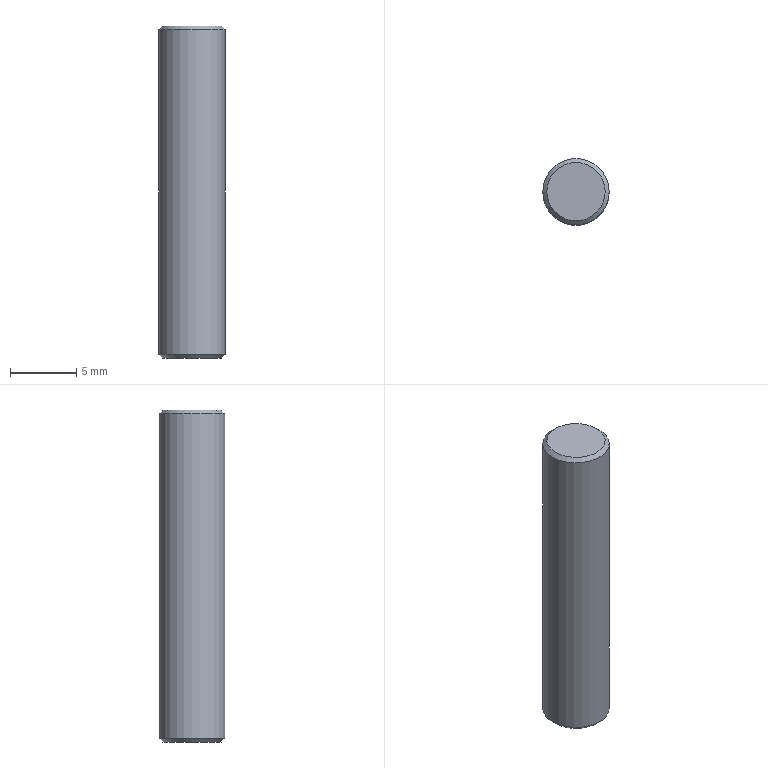Component | NX | DOWEL_PIN | 1 solid | 5 faces | box 5 x 5 x 25 mm | volume 490 mm3 | plane 2 | cone 2 | cylinder 1 | commonest cylinder face diameters 5 x1
STEP:
#1=CARTESIAN_POINT('',(0.,0.,0.));
#2=DIRECTION('',(0.,0.,1.));
#3=DIRECTION('',(1.,0.,0.));
#4=AXIS2_PLACEMENT_3D('',#1,#2,#3);
#5=CARTESIAN_POINT('',(96.2,25.,-225.));
#6=VERTEX_POINT('',#5);
#7=CARTESIAN_POINT('',(94.,25.,-225.));
#8=DIRECTION('',(0.,0.,1.));
#9=DIRECTION('',(1.,0.,0.));
#10=AXIS2_PLACEMENT_3D('',#7,#8,#9);
#11=CIRCLE('',#10,2.2);
#12=CARTESIAN_POINT('',(94.,25.,-225.));
#13=DIRECTION('',(0.,0.,1.));
#14=DIRECTION('',(1.,0.,0.));
#15=AXIS2_PLACEMENT_3D('',#12,#13,#14);
#16=PLANE('',#15);
#17=CARTESIAN_POINT('',(0.,0.));
#18=DIRECTION('',(1.,0.));
#19=AXIS2_PLACEMENT_2D('',#17,#18);
#20=CIRCLE('',#19,2.2);
#21=(GEOMETRIC_REPRESENTATION_CONTEXT(2)PARAMETRIC_REPRESENTATION_CONTEXT()REPRESENTATION_CONTEXT('',''));
#22=DEFINITIONAL_REPRESENTATION('',(#20),#21);
#23=PCURVE('',#16,#22);
#24=CARTESIAN_POINT('',(94.,25.,-225.3));
#25=DIRECTION('',(0.,0.,-1.));
#26=DIRECTION('',(-1.,0.,0.));
#27=AXIS2_PLACEMENT_3D('',#24,#25,#26);
#28=CONICAL_SURFACE('',#27,2.5,0.7854);
#29=CARTESIAN_POINT('',(9.425,-0.3));
#30=DIRECTION('',(-1.,0.));
#31=VECTOR('',#30,1.);
#32=LINE('',#29,#31);
#33=(GEOMETRIC_REPRESENTATION_CONTEXT(2)PARAMETRIC_REPRESENTATION_CONTEXT()REPRESENTATION_CONTEXT('',''));
#34=DEFINITIONAL_REPRESENTATION('',(#32),#33);
#35=PCURVE('',#28,#34);
#36=SURFACE_CURVE('',#11,(#23,#35),.PCURVE_S1.);
#37=EDGE_CURVE('',#6,#6,#36,.T.);
#38=ORIENTED_EDGE('',*,*,#37,.T.);
#39=EDGE_LOOP('',(#38));
#40=FACE_BOUND('',#39,.T.);
#41=ADVANCED_FACE('',(#40),#16,.T.);
#42=CARTESIAN_POINT('',(91.8,25.,-250.));
#43=VERTEX_POINT('',#42);
#44=CARTESIAN_POINT('',(94.,25.,-250.));
#45=DIRECTION('',(0.,0.,-1.));
#46=DIRECTION('',(-1.,0.,0.));
#47=AXIS2_PLACEMENT_3D('',#44,#45,#46);
#48=CIRCLE('',#47,2.2);
#49=CARTESIAN_POINT('',(94.,25.,-250.));
#50=DIRECTION('',(0.,0.,-1.));
#51=DIRECTION('',(-1.,0.,0.));
#52=AXIS2_PLACEMENT_3D('',#49,#50,#51);
#53=PLANE('',#52);
#54=CARTESIAN_POINT('',(0.,0.));
#55=DIRECTION('',(1.,0.));
#56=AXIS2_PLACEMENT_2D('',#54,#55);
#57=CIRCLE('',#56,2.2);
#58=(GEOMETRIC_REPRESENTATION_CONTEXT(2)PARAMETRIC_REPRESENTATION_CONTEXT()REPRESENTATION_CONTEXT('',''));
#59=DEFINITIONAL_REPRESENTATION('',(#57),#58);
#60=PCURVE('',#53,#59);
#61=CARTESIAN_POINT('',(94.,25.,-249.7));
#62=DIRECTION('',(0.,0.,1.));
#63=DIRECTION('',(1.,0.,0.));
#64=AXIS2_PLACEMENT_3D('',#61,#62,#63);
#65=CONICAL_SURFACE('',#64,2.5,0.7854);
#66=CARTESIAN_POINT('',(9.425,-0.3));
#67=DIRECTION('',(-1.,0.));
#68=VECTOR('',#67,1.);
#69=LINE('',#66,#68);
#70=(GEOMETRIC_REPRESENTATION_CONTEXT(2)PARAMETRIC_REPRESENTATION_CONTEXT()REPRESENTATION_CONTEXT('',''));
#71=DEFINITIONAL_REPRESENTATION('',(#69),#70);
#72=PCURVE('',#65,#71);
#73=SURFACE_CURVE('',#48,(#60,#72),.PCURVE_S1.);
#74=EDGE_CURVE('',#43,#43,#73,.T.);
#75=ORIENTED_EDGE('',*,*,#74,.T.);
#76=EDGE_LOOP('',(#75));
#77=FACE_BOUND('',#76,.T.);
#78=ADVANCED_FACE('',(#77),#53,.T.);
#79=CARTESIAN_POINT('',(91.5,25.,-249.7));
#80=VERTEX_POINT('',#79);
#81=CARTESIAN_POINT('',(96.5,25.,-249.7));
#82=VERTEX_POINT('',#81);
#83=CARTESIAN_POINT('',(94.,25.,-249.7));
#84=DIRECTION('',(0.,0.,1.));
#85=DIRECTION('',(-1.,0.,0.));
#86=AXIS2_PLACEMENT_3D('',#83,#84,#85);
#87=CIRCLE('',#86,2.5);
#88=CARTESIAN_POINT('',(94.,25.,-250.));
#89=DIRECTION('',(0.,0.,1.));
#90=DIRECTION('',(1.,0.,0.));
#91=AXIS2_PLACEMENT_3D('',#88,#89,#90);
#92=CYLINDRICAL_SURFACE('',#91,2.5);
#93=CARTESIAN_POINT('',(3.142,0.3));
#94=DIRECTION('',(1.,0.));
#95=VECTOR('',#94,1.);
#96=LINE('',#93,#95);
#97=(GEOMETRIC_REPRESENTATION_CONTEXT(2)PARAMETRIC_REPRESENTATION_CONTEXT()REPRESENTATION_CONTEXT('',''));
#98=DEFINITIONAL_REPRESENTATION('',(#96),#97);
#99=PCURVE('',#92,#98);
#100=CARTESIAN_POINT('',(3.142,0.));
#101=DIRECTION('',(1.,0.));
#102=VECTOR('',#101,1.);
#103=LINE('',#100,#102);
#104=(GEOMETRIC_REPRESENTATION_CONTEXT(2)PARAMETRIC_REPRESENTATION_CONTEXT()REPRESENTATION_CONTEXT('',''));
#105=DEFINITIONAL_REPRESENTATION('',(#103),#104);
#106=PCURVE('',#65,#105);
#107=SURFACE_CURVE('',#87,(#99,#106),.PCURVE_S1.);
#108=EDGE_CURVE('',#80,#82,#107,.T.);
#109=ORIENTED_EDGE('',*,*,#108,.T.);
#110=CARTESIAN_POINT('',(96.5,25.,-225.3));
#111=VERTEX_POINT('',#110);
#112=CARTESIAN_POINT('',(96.5,25.,-249.7));
#113=CARTESIAN_POINT('',(96.5,25.,-225.3));
#114=B_SPLINE_CURVE_WITH_KNOTS('',1,(#112,#113),.UNSPECIFIED.,.F.,.F.,(2,2),(0.3,24.7),.PIECEWISE_BEZIER_KNOTS.);
#115=CARTESIAN_POINT('',(6.283,0.));
#116=DIRECTION('',(0.,1.));
#117=VECTOR('',#116,1.);
#118=LINE('',#115,#117);
#119=(GEOMETRIC_REPRESENTATION_CONTEXT(2)PARAMETRIC_REPRESENTATION_CONTEXT()REPRESENTATION_CONTEXT('',''));
#120=DEFINITIONAL_REPRESENTATION('',(#118),#119);
#121=PCURVE('',#92,#120);
#122=CARTESIAN_POINT('',(0.,0.));
#123=DIRECTION('',(0.,1.));
#124=VECTOR('',#123,1.);
#125=LINE('',#122,#124);
#126=(GEOMETRIC_REPRESENTATION_CONTEXT(2)PARAMETRIC_REPRESENTATION_CONTEXT()REPRESENTATION_CONTEXT('',''));
#127=DEFINITIONAL_REPRESENTATION('',(#125),#126);
#128=PCURVE('',#92,#127);
#129=SEAM_CURVE('',#114,(#121,#128),.PCURVE_S1.);
#130=EDGE_CURVE('',#82,#111,#129,.T.);
#131=ORIENTED_EDGE('',*,*,#130,.T.);
#132=CARTESIAN_POINT('',(94.,25.,-225.3));
#133=DIRECTION('',(0.,0.,-1.));
#134=DIRECTION('',(1.,0.,0.));
#135=AXIS2_PLACEMENT_3D('',#132,#133,#134);
#136=CIRCLE('',#135,2.5);
#137=CARTESIAN_POINT('',(6.283,24.7));
#138=DIRECTION('',(-1.,0.));
#139=VECTOR('',#138,1.);
#140=LINE('',#137,#139);
#141=(GEOMETRIC_REPRESENTATION_CONTEXT(2)PARAMETRIC_REPRESENTATION_CONTEXT()REPRESENTATION_CONTEXT('',''));
#142=DEFINITIONAL_REPRESENTATION('',(#140),#141);
#143=PCURVE('',#92,#142);
#144=CARTESIAN_POINT('',(3.142,0.));
#145=DIRECTION('',(1.,0.));
#146=VECTOR('',#145,1.);
#147=LINE('',#144,#146);
#148=(GEOMETRIC_REPRESENTATION_CONTEXT(2)PARAMETRIC_REPRESENTATION_CONTEXT()REPRESENTATION_CONTEXT('',''));
#149=DEFINITIONAL_REPRESENTATION('',(#147),#148);
#150=PCURVE('',#28,#149);
#151=SURFACE_CURVE('',#136,(#143,#150),.PCURVE_S1.);
#152=EDGE_CURVE('',#111,#111,#151,.T.);
#153=ORIENTED_EDGE('',*,*,#152,.T.);
#154=ORIENTED_EDGE('',*,*,#130,.F.);
#155=CARTESIAN_POINT('',(94.,25.,-249.7));
#156=DIRECTION('',(0.,0.,1.));
#157=DIRECTION('',(-1.,0.,0.));
#158=AXIS2_PLACEMENT_3D('',#155,#156,#157);
#159=CIRCLE('',#158,2.5);
#160=CARTESIAN_POINT('',(-3.142,0.3));
#161=DIRECTION('',(1.,0.));
#162=VECTOR('',#161,1.);
#163=LINE('',#160,#162);
#164=(GEOMETRIC_REPRESENTATION_CONTEXT(2)PARAMETRIC_REPRESENTATION_CONTEXT()REPRESENTATION_CONTEXT('',''));
#165=DEFINITIONAL_REPRESENTATION('',(#163),#164);
#166=PCURVE('',#92,#165);
#167=CARTESIAN_POINT('',(3.142,0.));
#168=DIRECTION('',(1.,0.));
#169=VECTOR('',#168,1.);
#170=LINE('',#167,#169);
#171=(GEOMETRIC_REPRESENTATION_CONTEXT(2)PARAMETRIC_REPRESENTATION_CONTEXT()REPRESENTATION_CONTEXT('',''));
#172=DEFINITIONAL_REPRESENTATION('',(#170),#171);
#173=PCURVE('',#65,#172);
#174=SURFACE_CURVE('',#159,(#166,#173),.PCURVE_S1.);
#175=EDGE_CURVE('',#82,#80,#174,.T.);
#176=ORIENTED_EDGE('',*,*,#175,.T.);
#177=EDGE_LOOP('',(#109,#131,#153,#154,#176));
#178=FACE_BOUND('',#177,.T.);
#179=ADVANCED_FACE('',(#178),#92,.T.);
#180=ORIENTED_EDGE('',*,*,#74,.F.);
#181=CARTESIAN_POINT('',(91.8,25.,-250.));
#182=CARTESIAN_POINT('',(91.5,25.,-249.7));
#183=B_SPLINE_CURVE_WITH_KNOTS('',1,(#181,#182),.UNSPECIFIED.,.F.,.F.,(2,2),(-0.4243,0.),.PIECEWISE_BEZIER_KNOTS.);
#184=CARTESIAN_POINT('',(9.425,0.));
#185=DIRECTION('',(0.,1.));
#186=VECTOR('',#185,1.);
#187=LINE('',#184,#186);
#188=(GEOMETRIC_REPRESENTATION_CONTEXT(2)PARAMETRIC_REPRESENTATION_CONTEXT()REPRESENTATION_CONTEXT('',''));
#189=DEFINITIONAL_REPRESENTATION('',(#187),#188);
#190=PCURVE('',#65,#189);
#191=CARTESIAN_POINT('',(3.142,0.));
#192=DIRECTION('',(0.,1.));
#193=VECTOR('',#192,1.);
#194=LINE('',#191,#193);
#195=(GEOMETRIC_REPRESENTATION_CONTEXT(2)PARAMETRIC_REPRESENTATION_CONTEXT()REPRESENTATION_CONTEXT('',''));
#196=DEFINITIONAL_REPRESENTATION('',(#194),#195);
#197=PCURVE('',#65,#196);
#198=SEAM_CURVE('',#183,(#190,#197),.PCURVE_S1.);
#199=EDGE_CURVE('',#43,#80,#198,.T.);
#200=ORIENTED_EDGE('',*,*,#199,.T.);
#201=ORIENTED_EDGE('',*,*,#175,.F.);
#202=ORIENTED_EDGE('',*,*,#108,.F.);
#203=ORIENTED_EDGE('',*,*,#199,.F.);
#204=EDGE_LOOP('',(#180,#200,#201,#202,#203));
#205=FACE_BOUND('',#204,.T.);
#206=ADVANCED_FACE('',(#205),#65,.T.);
#207=ORIENTED_EDGE('',*,*,#37,.F.);
#208=CARTESIAN_POINT('',(96.2,25.,-225.));
#209=CARTESIAN_POINT('',(96.5,25.,-225.3));
#210=B_SPLINE_CURVE_WITH_KNOTS('',1,(#208,#209),.UNSPECIFIED.,.F.,.F.,(2,2),(-0.4243,0.),.PIECEWISE_BEZIER_KNOTS.);
#211=CARTESIAN_POINT('',(9.425,0.));
#212=DIRECTION('',(0.,1.));
#213=VECTOR('',#212,1.);
#214=LINE('',#211,#213);
#215=(GEOMETRIC_REPRESENTATION_CONTEXT(2)PARAMETRIC_REPRESENTATION_CONTEXT()REPRESENTATION_CONTEXT('',''));
#216=DEFINITIONAL_REPRESENTATION('',(#214),#215);
#217=PCURVE('',#28,#216);
#218=CARTESIAN_POINT('',(3.142,0.));
#219=DIRECTION('',(0.,1.));
#220=VECTOR('',#219,1.);
#221=LINE('',#218,#220);
#222=(GEOMETRIC_REPRESENTATION_CONTEXT(2)PARAMETRIC_REPRESENTATION_CONTEXT()REPRESENTATION_CONTEXT('',''));
#223=DEFINITIONAL_REPRESENTATION('',(#221),#222);
#224=PCURVE('',#28,#223);
#225=SEAM_CURVE('',#210,(#217,#224),.PCURVE_S1.);
#226=EDGE_CURVE('',#6,#111,#225,.T.);
#227=ORIENTED_EDGE('',*,*,#226,.T.);
#228=ORIENTED_EDGE('',*,*,#152,.F.);
#229=ORIENTED_EDGE('',*,*,#226,.F.);
#230=EDGE_LOOP('',(#207,#227,#228,#229));
#231=FACE_BOUND('',#230,.T.);
#232=ADVANCED_FACE('',(#231),#28,.T.);
#233=CLOSED_SHELL('',(#41,#78,#179,#206,#232));
#234=MANIFOLD_SOLID_BREP('',#233);
#235=(LENGTH_UNIT()NAMED_UNIT(*)SI_UNIT(.MILLI.,.METRE.));
#236=UNCERTAINTY_MEASURE_WITH_UNIT(LENGTH_MEASURE(0.00001),#235,'','');
#237=(NAMED_UNIT(*)PLANE_ANGLE_UNIT()SI_UNIT($,.RADIAN.));
#238=(NAMED_UNIT(*)SI_UNIT($,.STERADIAN.)SOLID_ANGLE_UNIT());
#239=(GEOMETRIC_REPRESENTATION_CONTEXT(3)GLOBAL_UNCERTAINTY_ASSIGNED_CONTEXT((#236))GLOBAL_UNIT_ASSIGNED_CONTEXT((#235,#237,#238))REPRESENTATION_CONTEXT('',''));
#240=ADVANCED_BREP_SHAPE_REPRESENTATION('',(#4,#234),#239);